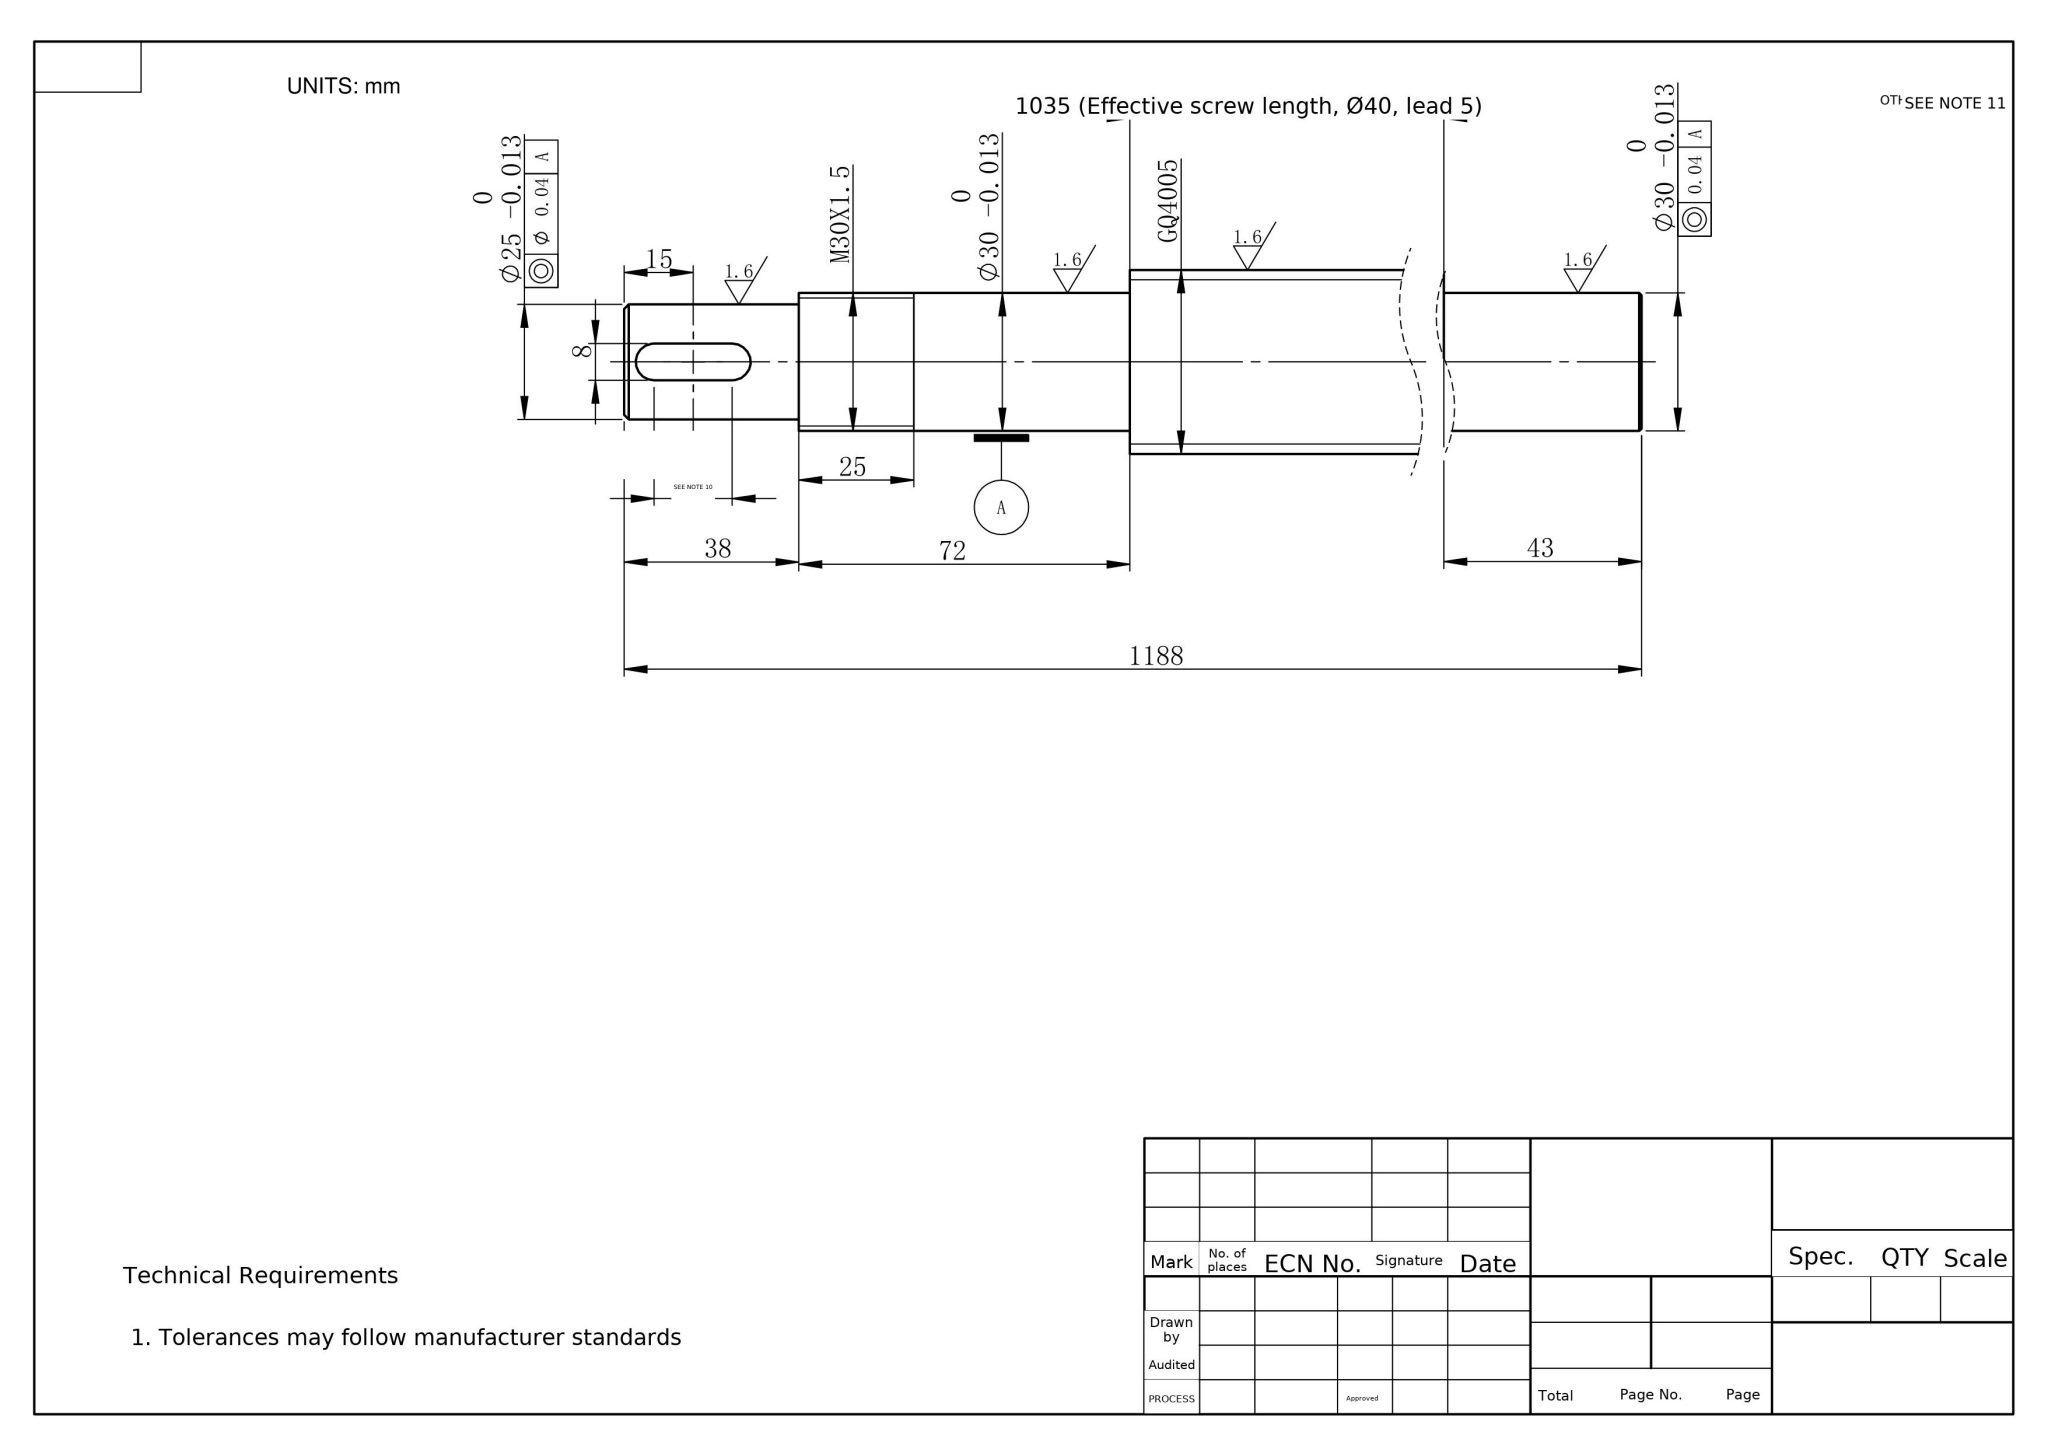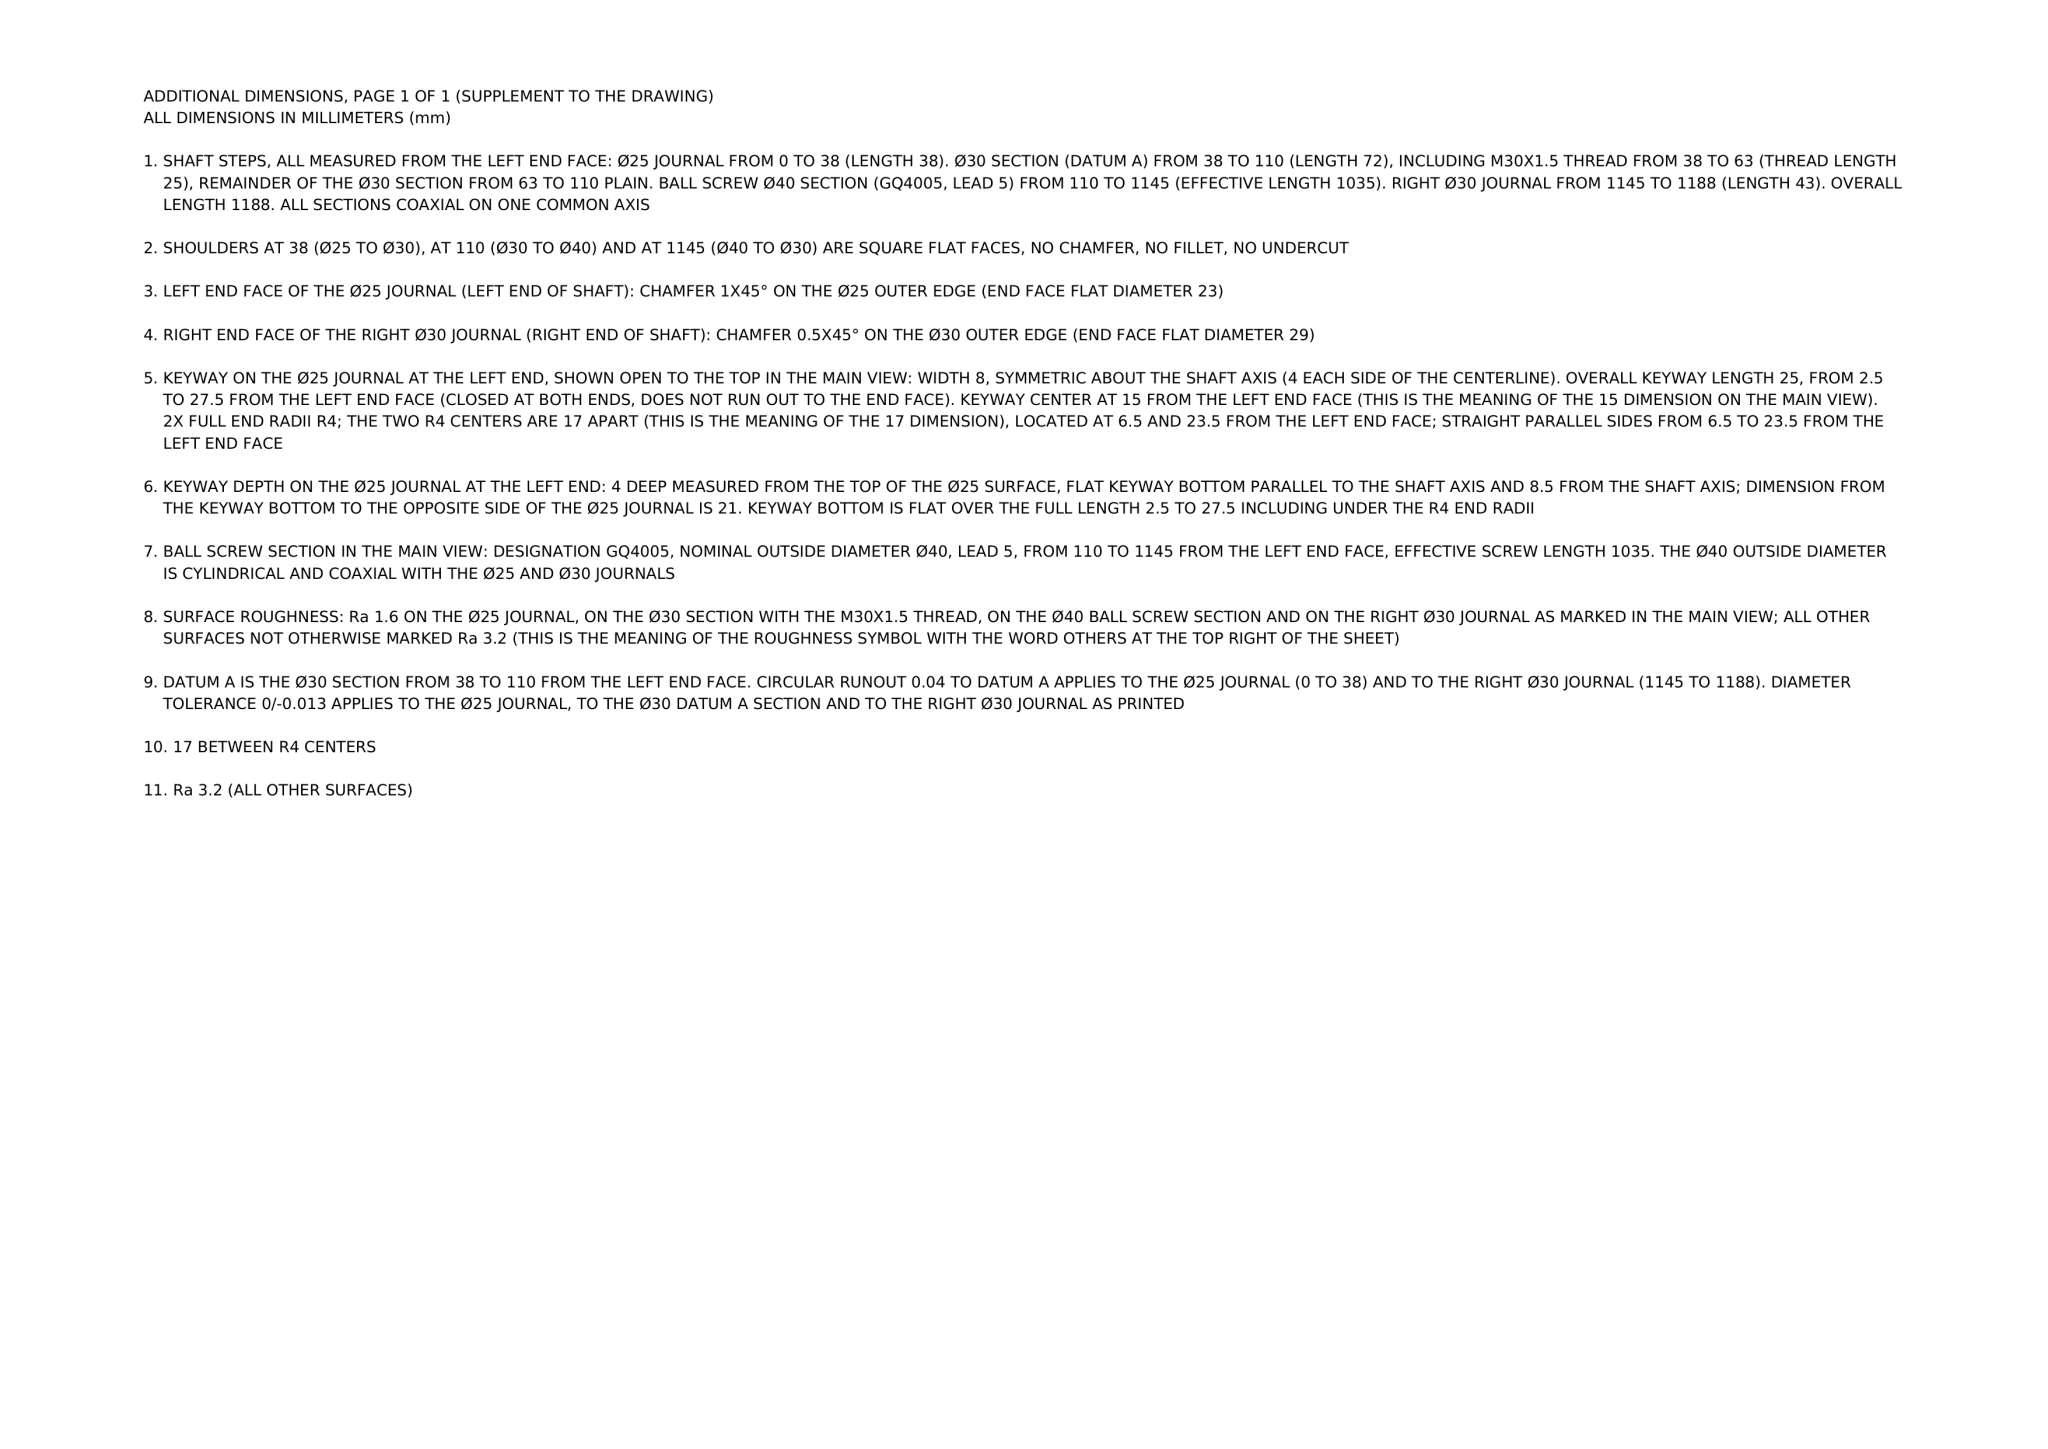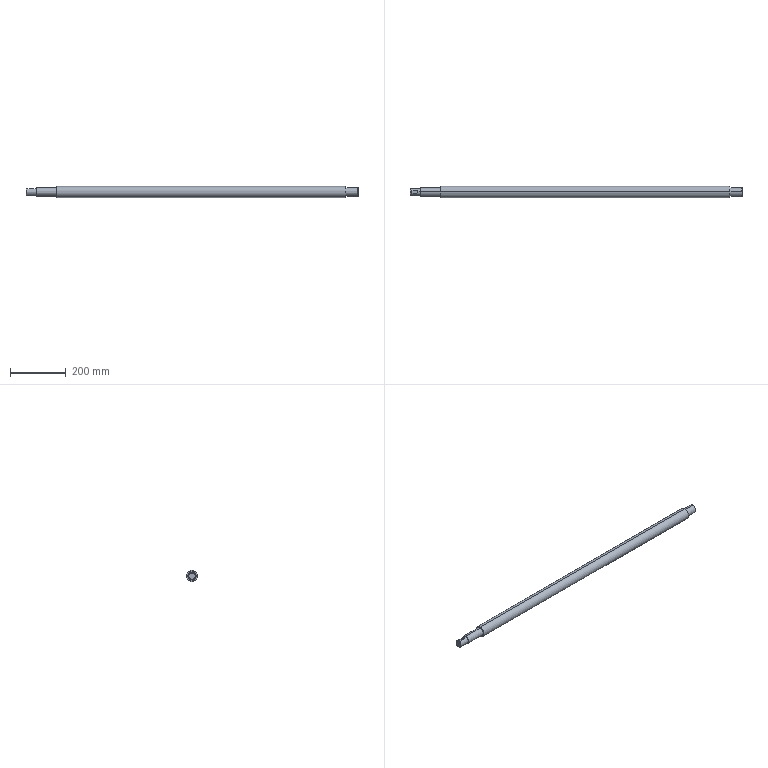Part | NX | mm | 1 solid | 23 faces | box 1188 x 40 x 40 mm | volume 1399804 mm3 | cylinder 11 | plane 8 | cone 4 | commonest cylinder face diameters 30 x4 8 x3 40 x2 25 x2
STEP:
#1=COLOUR_RGB('',1.,0.949,0.9098);
#2=FILL_AREA_STYLE_COLOUR('',#1);
#3=FILL_AREA_STYLE('',(#2));
#4=SURFACE_STYLE_FILL_AREA(#3);
#5=SURFACE_SIDE_STYLE('',(#4));
#6=SURFACE_STYLE_USAGE(.BOTH.,#5);
#7=PRESENTATION_STYLE_ASSIGNMENT((#6));
#8=CARTESIAN_POINT('',(110.,0.,-15.));
#9=VERTEX_POINT('',#8);
#10=CARTESIAN_POINT('',(38.,0.,-15.));
#11=VERTEX_POINT('',#10);
#12=CARTESIAN_POINT('',(0.,0.,-15.));
#13=DIRECTION('',(-1.,0.,0.));
#14=VECTOR('',#13,1000.);
#15=LINE('',#12,#14);
#16=EDGE_CURVE('',#9,#11,#15,.T.);
#17=ORIENTED_EDGE('',*,*,#16,.F.);
#18=CARTESIAN_POINT('',(110.,0.,15.));
#19=VERTEX_POINT('',#18);
#20=CARTESIAN_POINT('',(110.,0.,0.));
#21=DIRECTION('',(-1.,0.,0.));
#22=DIRECTION('',(0.,0.,1.));
#23=AXIS2_PLACEMENT_3D('',#20,#21,#22);
#24=CIRCLE('',#23,15.);
#25=EDGE_CURVE('',#9,#19,#24,.T.);
#26=ORIENTED_EDGE('',*,*,#25,.T.);
#27=CARTESIAN_POINT('',(38.,0.,15.));
#28=VERTEX_POINT('',#27);
#29=CARTESIAN_POINT('',(0.,0.,15.));
#30=DIRECTION('',(-1.,0.,0.));
#31=VECTOR('',#30,1000.);
#32=LINE('',#29,#31);
#33=EDGE_CURVE('',#19,#28,#32,.T.);
#34=ORIENTED_EDGE('',*,*,#33,.T.);
#35=CARTESIAN_POINT('',(38.,0.,0.));
#36=DIRECTION('',(-1.,0.,0.));
#37=DIRECTION('',(0.,0.,1.));
#38=AXIS2_PLACEMENT_3D('',#35,#36,#37);
#39=CIRCLE('',#38,15.);
#40=EDGE_CURVE('',#11,#28,#39,.T.);
#41=ORIENTED_EDGE('',*,*,#40,.F.);
#42=EDGE_LOOP('',(#17,#26,#34,#41));
#43=FACE_OUTER_BOUND('',#42,.T.);
#44=CARTESIAN_POINT('',(0.,0.,0.));
#45=DIRECTION('',(-1.,0.,0.));
#46=DIRECTION('',(0.,0.,1.));
#47=AXIS2_PLACEMENT_3D('',#44,#45,#46);
#48=CYLINDRICAL_SURFACE('',#47,15.);
#49=ADVANCED_FACE('',(#43),#48,.T.);
#50=STYLED_ITEM('',(#7),#49);
#51=(LENGTH_UNIT()NAMED_UNIT(*)SI_UNIT(.MILLI.,.METRE.));
#52=UNCERTAINTY_MEASURE_WITH_UNIT(LENGTH_MEASURE(0.00001),#51,'','');
#53=(NAMED_UNIT(*)PLANE_ANGLE_UNIT()SI_UNIT($,.RADIAN.));
#54=(NAMED_UNIT(*)SI_UNIT($,.STERADIAN.)SOLID_ANGLE_UNIT());
#55=(GEOMETRIC_REPRESENTATION_CONTEXT(3)GLOBAL_UNCERTAINTY_ASSIGNED_CONTEXT((#52))GLOBAL_UNIT_ASSIGNED_CONTEXT((#51,#53,#54))REPRESENTATION_CONTEXT('',''));
#56=MECHANICAL_DESIGN_GEOMETRIC_PRESENTATION_REPRESENTATION('',(#50),#55);
#57=PRESENTATION_LAYER_ASSIGNMENT('','',(#50));
#58=COLOUR_RGB('',1.,0.949,0.9098);
#59=FILL_AREA_STYLE_COLOUR('',#58);
#60=FILL_AREA_STYLE('',(#59));
#61=SURFACE_STYLE_FILL_AREA(#60);
#62=SURFACE_SIDE_STYLE('',(#61));
#63=SURFACE_STYLE_USAGE(.BOTH.,#62);
#64=PRESENTATION_STYLE_ASSIGNMENT((#63));
#65=CARTESIAN_POINT('',(1145.,0.,20.));
#66=VERTEX_POINT('',#65);
#67=CARTESIAN_POINT('',(1145.,0.,-20.));
#68=VERTEX_POINT('',#67);
#69=CARTESIAN_POINT('',(1145.,0.,0.));
#70=DIRECTION('',(-1.,0.,0.));
#71=DIRECTION('',(0.,0.,1.));
#72=AXIS2_PLACEMENT_3D('',#69,#70,#71);
#73=CIRCLE('',#72,20.);
#74=EDGE_CURVE('',#66,#68,#73,.T.);
#75=ORIENTED_EDGE('',*,*,#74,.T.);
#76=CARTESIAN_POINT('',(110.,0.,-20.));
#77=VERTEX_POINT('',#76);
#78=CARTESIAN_POINT('',(0.,0.,-20.));
#79=DIRECTION('',(-1.,0.,0.));
#80=VECTOR('',#79,1000.);
#81=LINE('',#78,#80);
#82=EDGE_CURVE('',#68,#77,#81,.T.);
#83=ORIENTED_EDGE('',*,*,#82,.T.);
#84=CARTESIAN_POINT('',(110.,0.,20.));
#85=VERTEX_POINT('',#84);
#86=CARTESIAN_POINT('',(110.,0.,0.));
#87=DIRECTION('',(-1.,0.,0.));
#88=DIRECTION('',(0.,0.,1.));
#89=AXIS2_PLACEMENT_3D('',#86,#87,#88);
#90=CIRCLE('',#89,20.);
#91=EDGE_CURVE('',#85,#77,#90,.T.);
#92=ORIENTED_EDGE('',*,*,#91,.F.);
#93=CARTESIAN_POINT('',(0.,0.,20.));
#94=DIRECTION('',(-1.,0.,0.));
#95=VECTOR('',#94,1000.);
#96=LINE('',#93,#95);
#97=EDGE_CURVE('',#66,#85,#96,.T.);
#98=ORIENTED_EDGE('',*,*,#97,.F.);
#99=EDGE_LOOP('',(#75,#83,#92,#98));
#100=FACE_OUTER_BOUND('',#99,.T.);
#101=CARTESIAN_POINT('',(0.,0.,0.));
#102=DIRECTION('',(-1.,0.,0.));
#103=DIRECTION('',(0.,0.,1.));
#104=AXIS2_PLACEMENT_3D('',#101,#102,#103);
#105=CYLINDRICAL_SURFACE('',#104,20.);
#106=ADVANCED_FACE('',(#100),#105,.T.);
#107=STYLED_ITEM('',(#64),#106);
#108=(LENGTH_UNIT()NAMED_UNIT(*)SI_UNIT(.MILLI.,.METRE.));
#109=UNCERTAINTY_MEASURE_WITH_UNIT(LENGTH_MEASURE(0.00001),#108,'','');
#110=(NAMED_UNIT(*)PLANE_ANGLE_UNIT()SI_UNIT($,.RADIAN.));
#111=(NAMED_UNIT(*)SI_UNIT($,.STERADIAN.)SOLID_ANGLE_UNIT());
#112=(GEOMETRIC_REPRESENTATION_CONTEXT(3)GLOBAL_UNCERTAINTY_ASSIGNED_CONTEXT((#109))GLOBAL_UNIT_ASSIGNED_CONTEXT((#108,#110,#111))REPRESENTATION_CONTEXT('',''));
#113=MECHANICAL_DESIGN_GEOMETRIC_PRESENTATION_REPRESENTATION('',(#107),#112);
#114=COLOUR_RGB('',1.,0.949,0.9098);
#115=FILL_AREA_STYLE_COLOUR('',#114);
#116=FILL_AREA_STYLE('',(#115));
#117=SURFACE_STYLE_FILL_AREA(#116);
#118=SURFACE_SIDE_STYLE('',(#117));
#119=SURFACE_STYLE_USAGE(.BOTH.,#118);
#120=PRESENTATION_STYLE_ASSIGNMENT((#119));
#121=ORIENTED_EDGE('',*,*,#82,.F.);
#122=CARTESIAN_POINT('',(1145.,0.,0.));
#123=DIRECTION('',(-1.,0.,0.));
#124=DIRECTION('',(0.,0.,1.));
#125=AXIS2_PLACEMENT_3D('',#122,#123,#124);
#126=CIRCLE('',#125,20.);
#127=EDGE_CURVE('',#68,#66,#126,.T.);
#128=ORIENTED_EDGE('',*,*,#127,.T.);
#129=ORIENTED_EDGE('',*,*,#97,.T.);
#130=CARTESIAN_POINT('',(110.,0.,0.));
#131=DIRECTION('',(-1.,0.,0.));
#132=DIRECTION('',(0.,0.,1.));
#133=AXIS2_PLACEMENT_3D('',#130,#131,#132);
#134=CIRCLE('',#133,20.);
#135=EDGE_CURVE('',#77,#85,#134,.T.);
#136=ORIENTED_EDGE('',*,*,#135,.F.);
#137=EDGE_LOOP('',(#121,#128,#129,#136));
#138=FACE_OUTER_BOUND('',#137,.T.);
#139=CARTESIAN_POINT('',(0.,0.,0.));
#140=DIRECTION('',(-1.,0.,0.));
#141=DIRECTION('',(0.,0.,1.));
#142=AXIS2_PLACEMENT_3D('',#139,#140,#141);
#143=CYLINDRICAL_SURFACE('',#142,20.);
#144=ADVANCED_FACE('',(#138),#143,.T.);
#145=STYLED_ITEM('',(#120),#144);
#146=(LENGTH_UNIT()NAMED_UNIT(*)SI_UNIT(.MILLI.,.METRE.));
#147=UNCERTAINTY_MEASURE_WITH_UNIT(LENGTH_MEASURE(0.00001),#146,'','');
#148=(NAMED_UNIT(*)PLANE_ANGLE_UNIT()SI_UNIT($,.RADIAN.));
#149=(NAMED_UNIT(*)SI_UNIT($,.STERADIAN.)SOLID_ANGLE_UNIT());
#150=(GEOMETRIC_REPRESENTATION_CONTEXT(3)GLOBAL_UNCERTAINTY_ASSIGNED_CONTEXT((#147))GLOBAL_UNIT_ASSIGNED_CONTEXT((#146,#148,#149))REPRESENTATION_CONTEXT('',''));
#151=MECHANICAL_DESIGN_GEOMETRIC_PRESENTATION_REPRESENTATION('',(#145),#150);
#152=PRESENTATION_LAYER_ASSIGNMENT('','',(#107));
#153=COLOUR_RGB('',1.,0.949,0.9098);
#154=FILL_AREA_STYLE_COLOUR('',#153);
#155=FILL_AREA_STYLE('',(#154));
#156=SURFACE_STYLE_FILL_AREA(#155);
#157=SURFACE_SIDE_STYLE('',(#156));
#158=SURFACE_STYLE_USAGE(.BOTH.,#157);
#159=PRESENTATION_STYLE_ASSIGNMENT((#158));
#160=CARTESIAN_POINT('',(27.5,0.,8.5));
#161=VERTEX_POINT('',#160);
#162=CARTESIAN_POINT('',(23.5,4.,8.5));
#163=VERTEX_POINT('',#162);
#164=CARTESIAN_POINT('',(23.5,0.,8.5));
#165=DIRECTION('',(0.,0.,1.));
#166=DIRECTION('',(1.,0.,0.));
#167=AXIS2_PLACEMENT_3D('',#164,#165,#166);
#168=CIRCLE('',#167,4.);
#169=EDGE_CURVE('',#161,#163,#168,.T.);
#170=ORIENTED_EDGE('',*,*,#169,.F.);
#171=CARTESIAN_POINT('',(27.5,0.,12.5));
#172=VERTEX_POINT('',#171);
#173=CARTESIAN_POINT('',(27.5,0.,8.5));
#174=DIRECTION('',(0.,0.,1.));
#175=VECTOR('',#174,1000.);
#176=LINE('',#173,#175);
#177=EDGE_CURVE('',#161,#172,#176,.T.);
#178=ORIENTED_EDGE('',*,*,#177,.T.);
#179=CARTESIAN_POINT('',(23.5,4.,11.843));
#180=VERTEX_POINT('',#179);
#181=CARTESIAN_POINT('',(23.5,4.,11.843));
#182=CARTESIAN_POINT('',(23.766,4.,11.843));
#183=CARTESIAN_POINT('',(24.028,3.974,11.852));
#184=CARTESIAN_POINT('',(24.541,3.871,11.886));
#185=CARTESIAN_POINT('',(24.796,3.793,11.911));
#186=CARTESIAN_POINT('',(25.28,3.592,11.973));
#187=CARTESIAN_POINT('',(25.509,3.469,12.01));
#188=CARTESIAN_POINT('',(25.943,3.178,12.09));
#189=CARTESIAN_POINT('',(26.146,3.011,12.134));
#190=CARTESIAN_POINT('',(26.513,2.644,12.219));
#191=CARTESIAN_POINT('',(26.678,2.444,12.261));
#192=CARTESIAN_POINT('',(26.97,2.006,12.34));
#193=CARTESIAN_POINT('',(27.093,1.776,12.375));
#194=CARTESIAN_POINT('',(27.293,1.295,12.435));
#195=CARTESIAN_POINT('',(27.371,1.041,12.459));
#196=CARTESIAN_POINT('',(27.474,0.5239,12.492));
#197=CARTESIAN_POINT('',(27.5,0.263,12.5));
#198=CARTESIAN_POINT('',(27.5,0.,12.5));
#199=B_SPLINE_CURVE_WITH_KNOTS('',3,(#181,#182,#183,#184,#185,#186,#187,#188,#189,#190,#191,#192,#193,#194,#195,#196,#197,#198),.UNSPECIFIED.,.F.,.F.,(4,2,2,2,2,2,2,2,4),(0.,0.000787,0.001574,0.002361,0.003148,0.003935,0.004722,0.005509,0.006296),.UNSPECIFIED.);
#200=EDGE_CURVE('',#180,#172,#199,.T.);
#201=ORIENTED_EDGE('',*,*,#200,.F.);
#202=CARTESIAN_POINT('',(23.5,4.,8.5));
#203=DIRECTION('',(0.,0.,1.));
#204=VECTOR('',#203,1000.);
#205=LINE('',#202,#204);
#206=EDGE_CURVE('',#163,#180,#205,.T.);
#207=ORIENTED_EDGE('',*,*,#206,.F.);
#208=EDGE_LOOP('',(#170,#178,#201,#207));
#209=FACE_OUTER_BOUND('',#208,.T.);
#210=CARTESIAN_POINT('',(23.5,0.,8.5));
#211=DIRECTION('',(0.,0.,1.));
#212=DIRECTION('',(1.,0.,0.));
#213=AXIS2_PLACEMENT_3D('',#210,#211,#212);
#214=CYLINDRICAL_SURFACE('',#213,4.);
#215=ADVANCED_FACE('',(#209),#214,.F.);
#216=CARTESIAN_POINT('',(1188.,0.,14.5));
#217=VERTEX_POINT('',#216);
#218=CARTESIAN_POINT('',(1188.,0.,-14.5));
#219=VERTEX_POINT('',#218);
#220=CARTESIAN_POINT('',(1188.,0.,0.));
#221=DIRECTION('',(-1.,0.,0.));
#222=DIRECTION('',(0.,0.,1.));
#223=AXIS2_PLACEMENT_3D('',#220,#221,#222);
#224=CIRCLE('',#223,14.5);
#225=EDGE_CURVE('',#217,#219,#224,.T.);
#226=ORIENTED_EDGE('',*,*,#225,.T.);
#227=CARTESIAN_POINT('',(1187.5,0.,-15.));
#228=VERTEX_POINT('',#227);
#229=CARTESIAN_POINT('',(1188.,0.,-14.5));
#230=DIRECTION('',(-0.7071,0.,-0.7071));
#231=VECTOR('',#230,1000.);
#232=LINE('',#229,#231);
#233=EDGE_CURVE('',#219,#228,#232,.T.);
#234=ORIENTED_EDGE('',*,*,#233,.T.);
#235=CARTESIAN_POINT('',(1187.5,0.,15.));
#236=VERTEX_POINT('',#235);
#237=CARTESIAN_POINT('',(1187.5,0.,0.));
#238=DIRECTION('',(-1.,0.,0.));
#239=DIRECTION('',(0.,0.,1.));
#240=AXIS2_PLACEMENT_3D('',#237,#238,#239);
#241=CIRCLE('',#240,15.);
#242=EDGE_CURVE('',#236,#228,#241,.T.);
#243=ORIENTED_EDGE('',*,*,#242,.F.);
#244=CARTESIAN_POINT('',(1188.,0.,14.5));
#245=DIRECTION('',(-0.7071,0.,0.7071));
#246=VECTOR('',#245,1000.);
#247=LINE('',#244,#246);
#248=EDGE_CURVE('',#217,#236,#247,.T.);
#249=ORIENTED_EDGE('',*,*,#248,.F.);
#250=EDGE_LOOP('',(#226,#234,#243,#249));
#251=FACE_OUTER_BOUND('',#250,.T.);
#252=CARTESIAN_POINT('',(1188.,0.,0.));
#253=DIRECTION('',(-1.,0.,0.));
#254=DIRECTION('',(0.,0.,1.));
#255=AXIS2_PLACEMENT_3D('',#252,#253,#254);
#256=CONICAL_SURFACE('',#255,14.5,0.7854);
#257=ADVANCED_FACE('',(#251),#256,.T.);
#258=ORIENTED_EDGE('',*,*,#242,.T.);
#259=CARTESIAN_POINT('',(1145.,0.,-15.));
#260=VERTEX_POINT('',#259);
#261=CARTESIAN_POINT('',(0.,0.,-15.));
#262=DIRECTION('',(-1.,0.,0.));
#263=VECTOR('',#262,1000.);
#264=LINE('',#261,#263);
#265=EDGE_CURVE('',#228,#260,#264,.T.);
#266=ORIENTED_EDGE('',*,*,#265,.T.);
#267=CARTESIAN_POINT('',(1145.,0.,15.));
#268=VERTEX_POINT('',#267);
#269=CARTESIAN_POINT('',(1145.,0.,0.));
#270=DIRECTION('',(-1.,0.,0.));
#271=DIRECTION('',(0.,0.,1.));
#272=AXIS2_PLACEMENT_3D('',#269,#270,#271);
#273=CIRCLE('',#272,15.);
#274=EDGE_CURVE('',#268,#260,#273,.T.);
#275=ORIENTED_EDGE('',*,*,#274,.F.);
#276=CARTESIAN_POINT('',(0.,0.,15.));
#277=DIRECTION('',(-1.,0.,0.));
#278=VECTOR('',#277,1000.);
#279=LINE('',#276,#278);
#280=EDGE_CURVE('',#236,#268,#279,.T.);
#281=ORIENTED_EDGE('',*,*,#280,.F.);
#282=EDGE_LOOP('',(#258,#266,#275,#281));
#283=FACE_OUTER_BOUND('',#282,.T.);
#284=CARTESIAN_POINT('',(0.,0.,0.));
#285=DIRECTION('',(-1.,0.,0.));
#286=DIRECTION('',(0.,0.,1.));
#287=AXIS2_PLACEMENT_3D('',#284,#285,#286);
#288=CYLINDRICAL_SURFACE('',#287,15.);
#289=ADVANCED_FACE('',(#283),#288,.T.);
#290=CARTESIAN_POINT('',(110.,0.,0.));
#291=DIRECTION('',(-1.,0.,0.));
#292=DIRECTION('',(0.,0.,1.));
#293=AXIS2_PLACEMENT_3D('',#290,#291,#292);
#294=CIRCLE('',#293,15.);
#295=EDGE_CURVE('',#19,#9,#294,.T.);
#296=ORIENTED_EDGE('',*,*,#295,.T.);
#297=ORIENTED_EDGE('',*,*,#16,.T.);
#298=CARTESIAN_POINT('',(38.,0.,0.));
#299=DIRECTION('',(-1.,0.,0.));
#300=DIRECTION('',(0.,0.,1.));
#301=AXIS2_PLACEMENT_3D('',#298,#299,#300);
#302=CIRCLE('',#301,15.);
#303=EDGE_CURVE('',#28,#11,#302,.T.);
#304=ORIENTED_EDGE('',*,*,#303,.F.);
#305=ORIENTED_EDGE('',*,*,#33,.F.);
#306=EDGE_LOOP('',(#296,#297,#304,#305));
#307=FACE_OUTER_BOUND('',#306,.T.);
#308=CARTESIAN_POINT('',(0.,0.,0.));
#309=DIRECTION('',(-1.,0.,0.));
#310=DIRECTION('',(0.,0.,1.));
#311=AXIS2_PLACEMENT_3D('',#308,#309,#310);
#312=CYLINDRICAL_SURFACE('',#311,15.);
#313=ADVANCED_FACE('',(#307),#312,.T.);
#314=CARTESIAN_POINT('',(38.,0.,12.5));
#315=VERTEX_POINT('',#314);
#316=CARTESIAN_POINT('',(38.,0.,-12.5));
#317=VERTEX_POINT('',#316);
#318=CARTESIAN_POINT('',(38.,0.,0.));
#319=DIRECTION('',(-1.,0.,0.));
#320=DIRECTION('',(0.,0.,1.));
#321=AXIS2_PLACEMENT_3D('',#318,#319,#320);
#322=CIRCLE('',#321,12.5);
#323=EDGE_CURVE('',#315,#317,#322,.T.);
#324=ORIENTED_EDGE('',*,*,#323,.T.);
#325=CARTESIAN_POINT('',(1.,0.,-12.5));
#326=VERTEX_POINT('',#325);
#327=CARTESIAN_POINT('',(0.,0.,-12.5));
#328=DIRECTION('',(-1.,0.,0.));
#329=VECTOR('',#328,1000.);
#330=LINE('',#327,#329);
#331=EDGE_CURVE('',#317,#326,#330,.T.);
#332=ORIENTED_EDGE('',*,*,#331,.T.);
#333=CARTESIAN_POINT('',(1.,0.,12.5));
#334=VERTEX_POINT('',#333);
#335=CARTESIAN_POINT('',(1.,0.,0.));
#336=DIRECTION('',(-1.,0.,0.));
#337=DIRECTION('',(0.,0.,1.));
#338=AXIS2_PLACEMENT_3D('',#335,#336,#337);
#339=CIRCLE('',#338,12.5);
#340=EDGE_CURVE('',#334,#326,#339,.T.);
#341=ORIENTED_EDGE('',*,*,#340,.F.);
#342=CARTESIAN_POINT('',(2.5,-0.,12.5));
#343=VERTEX_POINT('',#342);
#344=CARTESIAN_POINT('',(0.,0.,12.5));
#345=DIRECTION('',(-1.,0.,0.));
#346=VECTOR('',#345,1000.);
#347=LINE('',#344,#346);
#348=EDGE_CURVE('',#343,#334,#347,.T.);
#349=ORIENTED_EDGE('',*,*,#348,.F.);
#350=CARTESIAN_POINT('',(6.5,4.,11.843));
#351=VERTEX_POINT('',#350);
#352=CARTESIAN_POINT('',(2.5,-0.,12.5));
#353=CARTESIAN_POINT('',(2.5,0.2627,12.5));
#354=CARTESIAN_POINT('',(2.527,0.5294,12.491));
#355=CARTESIAN_POINT('',(2.63,1.043,12.459));
#356=CARTESIAN_POINT('',(2.706,1.293,12.435));
#357=CARTESIAN_POINT('',(2.908,1.78,12.375));
#358=CARTESIAN_POINT('',(3.032,2.011,12.339));
#359=CARTESIAN_POINT('',(3.321,2.442,12.261));
#360=CARTESIAN_POINT('',(3.488,2.645,12.218));
#361=CARTESIAN_POINT('',(3.856,3.013,12.133));
#362=CARTESIAN_POINT('',(4.056,3.177,12.09));
#363=CARTESIAN_POINT('',(4.488,3.467,12.011));
#364=CARTESIAN_POINT('',(4.722,3.592,11.973));
#365=CARTESIAN_POINT('',(5.203,3.793,11.911));
#366=CARTESIAN_POINT('',(5.452,3.869,11.886));
#367=CARTESIAN_POINT('',(5.968,3.973,11.852));
#368=CARTESIAN_POINT('',(6.234,4.,11.843));
#369=CARTESIAN_POINT('',(6.5,4.,11.843));
#370=B_SPLINE_CURVE_WITH_KNOTS('',3,(#352,#353,#354,#355,#356,#357,#358,#359,#360,#361,#362,#363,#364,#365,#366,#367,#368,#369),.UNSPECIFIED.,.F.,.F.,(4,2,2,2,2,2,2,2,4),(0.006296,0.007082,0.007868,0.008654,0.00944,0.01023,0.01101,0.0118,0.01258),.UNSPECIFIED.);
#371=EDGE_CURVE('',#343,#351,#370,.T.);
#372=ORIENTED_EDGE('',*,*,#371,.T.);
#373=CARTESIAN_POINT('',(-0.,4.,11.843));
#374=DIRECTION('',(1.,0.,0.));
#375=VECTOR('',#374,1000.);
#376=LINE('',#373,#375);
#377=EDGE_CURVE('',#351,#180,#376,.T.);
#378=ORIENTED_EDGE('',*,*,#377,.T.);
#379=ORIENTED_EDGE('',*,*,#200,.T.);
#380=CARTESIAN_POINT('',(0.,0.,12.5));
#381=DIRECTION('',(-1.,0.,0.));
#382=VECTOR('',#381,1000.);
#383=LINE('',#380,#382);
#384=EDGE_CURVE('',#315,#172,#383,.T.);
#385=ORIENTED_EDGE('',*,*,#384,.F.);
#386=EDGE_LOOP('',(#324,#332,#341,#349,#372,#378,#379,#385));
#387=FACE_OUTER_BOUND('',#386,.T.);
#388=CARTESIAN_POINT('',(0.,0.,0.));
#389=DIRECTION('',(-1.,0.,0.));
#390=DIRECTION('',(0.,0.,1.));
#391=AXIS2_PLACEMENT_3D('',#388,#389,#390);
#392=CYLINDRICAL_SURFACE('',#391,12.5);
#393=ADVANCED_FACE('',(#387),#392,.T.);
#394=CARTESIAN_POINT('',(0.,0.,11.5));
#395=VERTEX_POINT('',#394);
#396=CARTESIAN_POINT('',(0.,0.,-11.5));
#397=VERTEX_POINT('',#396);
#398=CARTESIAN_POINT('',(0.,0.,0.));
#399=DIRECTION('',(-1.,0.,0.));
#400=DIRECTION('',(0.,0.,1.));
#401=AXIS2_PLACEMENT_3D('',#398,#399,#400);
#402=CIRCLE('',#401,11.5);
#403=EDGE_CURVE('',#395,#397,#402,.T.);
#404=ORIENTED_EDGE('',*,*,#403,.F.);
#405=CARTESIAN_POINT('',(1.,0.,12.5));
#406=DIRECTION('',(0.7071,0.,0.7071));
#407=VECTOR('',#406,1000.);
#408=LINE('',#405,#407);
#409=EDGE_CURVE('',#395,#334,#408,.T.);
#410=ORIENTED_EDGE('',*,*,#409,.T.);
#411=ORIENTED_EDGE('',*,*,#340,.T.);
#412=CARTESIAN_POINT('',(1.,0.,-12.5));
#413=DIRECTION('',(0.7071,0.,-0.7071));
#414=VECTOR('',#413,1000.);
#415=LINE('',#412,#414);
#416=EDGE_CURVE('',#397,#326,#415,.T.);
#417=ORIENTED_EDGE('',*,*,#416,.F.);
#418=EDGE_LOOP('',(#404,#410,#411,#417));
#419=FACE_OUTER_BOUND('',#418,.T.);
#420=CARTESIAN_POINT('',(1.,0.,0.));
#421=DIRECTION('',(1.,0.,0.));
#422=DIRECTION('',(0.,0.,-1.));
#423=AXIS2_PLACEMENT_3D('',#420,#421,#422);
#424=CONICAL_SURFACE('',#423,12.5,0.7854);
#425=ADVANCED_FACE('',(#419),#424,.T.);
#426=CARTESIAN_POINT('',(0.,0.,0.));
#427=DIRECTION('',(-1.,0.,0.));
#428=DIRECTION('',(0.,0.,1.));
#429=AXIS2_PLACEMENT_3D('',#426,#427,#428);
#430=CIRCLE('',#429,11.5);
#431=EDGE_CURVE('',#397,#395,#430,.T.);
#432=ORIENTED_EDGE('',*,*,#431,.T.);
#433=ORIENTED_EDGE('',*,*,#403,.T.);
#434=EDGE_LOOP('',(#432,#433));
#435=FACE_OUTER_BOUND('',#434,.T.);
#436=CARTESIAN_POINT('',(0.,0.,0.));
#437=DIRECTION('',(1.,0.,0.));
#438=DIRECTION('',(0.,0.,-1.));
#439=AXIS2_PLACEMENT_3D('',#436,#437,#438);
#440=PLANE('',#439);
#441=ADVANCED_FACE('',(#435),#440,.F.);
#442=ORIENTED_EDGE('',*,*,#409,.F.);
#443=ORIENTED_EDGE('',*,*,#431,.F.);
#444=ORIENTED_EDGE('',*,*,#416,.T.);
#445=CARTESIAN_POINT('',(1.,0.,0.));
#446=DIRECTION('',(-1.,0.,0.));
#447=DIRECTION('',(0.,0.,1.));
#448=AXIS2_PLACEMENT_3D('',#445,#446,#447);
#449=CIRCLE('',#448,12.5);
#450=EDGE_CURVE('',#326,#334,#449,.T.);
#451=ORIENTED_EDGE('',*,*,#450,.T.);
#452=EDGE_LOOP('',(#442,#443,#444,#451));
#453=FACE_OUTER_BOUND('',#452,.T.);
#454=CARTESIAN_POINT('',(1.,0.,0.));
#455=DIRECTION('',(1.,0.,0.));
#456=DIRECTION('',(0.,0.,-1.));
#457=AXIS2_PLACEMENT_3D('',#454,#455,#456);
#458=CONICAL_SURFACE('',#457,12.5,0.7854);
#459=ADVANCED_FACE('',(#453),#458,.T.);
#460=ORIENTED_EDGE('',*,*,#331,.F.);
#461=CARTESIAN_POINT('',(38.,0.,0.));
#462=DIRECTION('',(-1.,0.,0.));
#463=DIRECTION('',(0.,0.,1.));
#464=AXIS2_PLACEMENT_3D('',#461,#462,#463);
#465=CIRCLE('',#464,12.5);
#466=EDGE_CURVE('',#317,#315,#465,.T.);
#467=ORIENTED_EDGE('',*,*,#466,.T.);
#468=ORIENTED_EDGE('',*,*,#384,.T.);
#469=CARTESIAN_POINT('',(23.5,-4.,11.843));
#470=VERTEX_POINT('',#469);
#471=CARTESIAN_POINT('',(27.5,0.,12.5));
#472=CARTESIAN_POINT('',(27.5,-0.2627,12.5));
#473=CARTESIAN_POINT('',(27.473,-0.5294,12.491));
#474=CARTESIAN_POINT('',(27.37,-1.043,12.459));
#475=CARTESIAN_POINT('',(27.294,-1.293,12.435));
#476=CARTESIAN_POINT('',(27.092,-1.78,12.375));
#477=CARTESIAN_POINT('',(26.968,-2.011,12.339));
#478=CARTESIAN_POINT('',(26.679,-2.442,12.261));
#479=CARTESIAN_POINT('',(26.512,-2.645,12.218));
#480=CARTESIAN_POINT('',(26.144,-3.013,12.133));
#481=CARTESIAN_POINT('',(25.944,-3.177,12.09));
#482=CARTESIAN_POINT('',(25.512,-3.467,12.011));
#483=CARTESIAN_POINT('',(25.278,-3.592,11.973));
#484=CARTESIAN_POINT('',(24.797,-3.793,11.911));
#485=CARTESIAN_POINT('',(24.548,-3.869,11.886));
#486=CARTESIAN_POINT('',(24.032,-3.973,11.852));
#487=CARTESIAN_POINT('',(23.766,-4.,11.843));
#488=CARTESIAN_POINT('',(23.5,-4.,11.843));
#489=B_SPLINE_CURVE_WITH_KNOTS('',3,(#471,#472,#473,#474,#475,#476,#477,#478,#479,#480,#481,#482,#483,#484,#485,#486,#487,#488),.UNSPECIFIED.,.F.,.F.,(4,2,2,2,2,2,2,2,4),(0.006296,0.007082,0.007868,0.008654,0.00944,0.01023,0.01101,0.0118,0.01258),.UNSPECIFIED.);
#490=EDGE_CURVE('',#172,#470,#489,.T.);
#491=ORIENTED_EDGE('',*,*,#490,.T.);
#492=CARTESIAN_POINT('',(6.5,-4.,11.843));
#493=VERTEX_POINT('',#492);
#494=CARTESIAN_POINT('',(0.,-4.,11.843));
#495=DIRECTION('',(-1.,0.,0.));
#496=VECTOR('',#495,1000.);
#497=LINE('',#494,#496);
#498=EDGE_CURVE('',#470,#493,#497,.T.);
#499=ORIENTED_EDGE('',*,*,#498,.T.);
#500=CARTESIAN_POINT('',(6.5,-4.,11.843));
#501=CARTESIAN_POINT('',(6.234,-4.,11.843));
#502=CARTESIAN_POINT('',(5.972,-3.974,11.852));
#503=CARTESIAN_POINT('',(5.459,-3.871,11.886));
#504=CARTESIAN_POINT('',(5.204,-3.793,11.911));
#505=CARTESIAN_POINT('',(4.72,-3.592,11.973));
#506=CARTESIAN_POINT('',(4.491,-3.469,12.01));
#507=CARTESIAN_POINT('',(4.057,-3.178,12.09));
#508=CARTESIAN_POINT('',(3.854,-3.011,12.134));
#509=CARTESIAN_POINT('',(3.487,-2.644,12.219));
#510=CARTESIAN_POINT('',(3.322,-2.444,12.261));
#511=CARTESIAN_POINT('',(3.03,-2.006,12.34));
#512=CARTESIAN_POINT('',(2.907,-1.776,12.375));
#513=CARTESIAN_POINT('',(2.707,-1.295,12.435));
#514=CARTESIAN_POINT('',(2.629,-1.041,12.459));
#515=CARTESIAN_POINT('',(2.526,-0.5239,12.492));
#516=CARTESIAN_POINT('',(2.5,-0.263,12.5));
#517=CARTESIAN_POINT('',(2.5,-0.,12.5));
#518=B_SPLINE_CURVE_WITH_KNOTS('',3,(#500,#501,#502,#503,#504,#505,#506,#507,#508,#509,#510,#511,#512,#513,#514,#515,#516,#517),.UNSPECIFIED.,.F.,.F.,(4,2,2,2,2,2,2,2,4),(0.,0.000787,0.001574,0.002361,0.003148,0.003935,0.004722,0.005509,0.006296),.UNSPECIFIED.);
#519=EDGE_CURVE('',#493,#343,#518,.T.);
#520=ORIENTED_EDGE('',*,*,#519,.T.);
#521=ORIENTED_EDGE('',*,*,#348,.T.);
#522=ORIENTED_EDGE('',*,*,#450,.F.);
#523=EDGE_LOOP('',(#460,#467,#468,#491,#499,#520,#521,#522));
#524=FACE_OUTER_BOUND('',#523,.T.);
#525=CARTESIAN_POINT('',(0.,0.,0.));
#526=DIRECTION('',(-1.,0.,0.));
#527=DIRECTION('',(0.,0.,1.));
#528=AXIS2_PLACEMENT_3D('',#525,#526,#527);
#529=CYLINDRICAL_SURFACE('',#528,12.5);
#530=ADVANCED_FACE('',(#524),#529,.T.);
#531=ORIENTED_EDGE('',*,*,#323,.F.);
#532=ORIENTED_EDGE('',*,*,#466,.F.);
#533=EDGE_LOOP('',(#531,#532));
#534=FACE_BOUND('',#533,.T.);
#535=ORIENTED_EDGE('',*,*,#303,.T.);
#536=ORIENTED_EDGE('',*,*,#40,.T.);
#537=EDGE_LOOP('',(#535,#536));
#538=FACE_OUTER_BOUND('',#537,.T.);
#539=CARTESIAN_POINT('',(38.,12.5,0.));
#540=DIRECTION('',(1.,0.,0.));
#541=DIRECTION('',(0.,0.,-1.));
#542=AXIS2_PLACEMENT_3D('',#539,#540,#541);
#543=PLANE('',#542);
#544=ADVANCED_FACE('',(#534,#538),#543,.F.);
#545=ORIENTED_EDGE('',*,*,#295,.F.);
#546=ORIENTED_EDGE('',*,*,#25,.F.);
#547=EDGE_LOOP('',(#545,#546));
#548=FACE_BOUND('',#547,.T.);
#549=ORIENTED_EDGE('',*,*,#91,.T.);
#550=ORIENTED_EDGE('',*,*,#135,.T.);
#551=EDGE_LOOP('',(#549,#550));
#552=FACE_OUTER_BOUND('',#551,.T.);
#553=CARTESIAN_POINT('',(110.,15.,0.));
#554=DIRECTION('',(1.,0.,0.));
#555=DIRECTION('',(0.,0.,-1.));
#556=AXIS2_PLACEMENT_3D('',#553,#554,#555);
#557=PLANE('',#556);
#558=ADVANCED_FACE('',(#548,#552),#557,.F.);
#559=ORIENTED_EDGE('',*,*,#74,.F.);
#560=ORIENTED_EDGE('',*,*,#127,.F.);
#561=EDGE_LOOP('',(#559,#560));
#562=FACE_OUTER_BOUND('',#561,.T.);
#563=ORIENTED_EDGE('',*,*,#274,.T.);
#564=CARTESIAN_POINT('',(1145.,0.,0.));
#565=DIRECTION('',(-1.,0.,0.));
#566=DIRECTION('',(0.,0.,1.));
#567=AXIS2_PLACEMENT_3D('',#564,#565,#566);
#568=CIRCLE('',#567,15.);
#569=EDGE_CURVE('',#260,#268,#568,.T.);
#570=ORIENTED_EDGE('',*,*,#569,.T.);
#571=EDGE_LOOP('',(#563,#570));
#572=FACE_BOUND('',#571,.T.);
#573=CARTESIAN_POINT('',(1145.,20.,0.));
#574=DIRECTION('',(-1.,0.,0.));
#575=DIRECTION('',(0.,0.,1.));
#576=AXIS2_PLACEMENT_3D('',#573,#574,#575);
#577=PLANE('',#576);
#578=ADVANCED_FACE('',(#562,#572),#577,.F.);
#579=ORIENTED_EDGE('',*,*,#265,.F.);
#580=CARTESIAN_POINT('',(1187.5,0.,0.));
#581=DIRECTION('',(-1.,0.,0.));
#582=DIRECTION('',(0.,0.,1.));
#583=AXIS2_PLACEMENT_3D('',#580,#581,#582);
#584=CIRCLE('',#583,15.);
#585=EDGE_CURVE('',#228,#236,#584,.T.);
#586=ORIENTED_EDGE('',*,*,#585,.T.);
#587=ORIENTED_EDGE('',*,*,#280,.T.);
#588=ORIENTED_EDGE('',*,*,#569,.F.);
#589=EDGE_LOOP('',(#579,#586,#587,#588));
#590=FACE_OUTER_BOUND('',#589,.T.);
#591=CARTESIAN_POINT('',(0.,0.,0.));
#592=DIRECTION('',(-1.,0.,0.));
#593=DIRECTION('',(0.,0.,1.));
#594=AXIS2_PLACEMENT_3D('',#591,#592,#593);
#595=CYLINDRICAL_SURFACE('',#594,15.);
#596=ADVANCED_FACE('',(#590),#595,.T.);
#597=ORIENTED_EDGE('',*,*,#233,.F.);
#598=CARTESIAN_POINT('',(1188.,0.,0.));
#599=DIRECTION('',(-1.,0.,0.));
#600=DIRECTION('',(0.,0.,1.));
#601=AXIS2_PLACEMENT_3D('',#598,#599,#600);
#602=CIRCLE('',#601,14.5);
#603=EDGE_CURVE('',#219,#217,#602,.T.);
#604=ORIENTED_EDGE('',*,*,#603,.T.);
#605=ORIENTED_EDGE('',*,*,#248,.T.);
#606=ORIENTED_EDGE('',*,*,#585,.F.);
#607=EDGE_LOOP('',(#597,#604,#605,#606));
#608=FACE_OUTER_BOUND('',#607,.T.);
#609=CARTESIAN_POINT('',(1188.,0.,0.));
#610=DIRECTION('',(-1.,0.,0.));
#611=DIRECTION('',(0.,0.,1.));
#612=AXIS2_PLACEMENT_3D('',#609,#610,#611);
#613=CONICAL_SURFACE('',#612,14.5,0.7854);
#614=ADVANCED_FACE('',(#608),#613,.T.);
#615=ORIENTED_EDGE('',*,*,#225,.F.);
#616=ORIENTED_EDGE('',*,*,#603,.F.);
#617=EDGE_LOOP('',(#615,#616));
#618=FACE_OUTER_BOUND('',#617,.T.);
#619=CARTESIAN_POINT('',(1188.,14.5,0.));
#620=DIRECTION('',(-1.,0.,0.));
#621=DIRECTION('',(0.,0.,1.));
#622=AXIS2_PLACEMENT_3D('',#619,#620,#621);
#623=PLANE('',#622);
#624=ADVANCED_FACE('',(#618),#623,.F.);
#625=CARTESIAN_POINT('',(6.5,-4.,8.5));
#626=VERTEX_POINT('',#625);
#627=CARTESIAN_POINT('',(6.5,-4.,8.5));
#628=DIRECTION('',(0.,0.,1.));
#629=VECTOR('',#628,1000.);
#630=LINE('',#627,#629);
#631=EDGE_CURVE('',#626,#493,#630,.T.);
#632=ORIENTED_EDGE('',*,*,#631,.F.);
#633=CARTESIAN_POINT('',(6.5,4.,8.5));
#634=VERTEX_POINT('',#633);
#635=CARTESIAN_POINT('',(6.5,0.,8.5));
#636=DIRECTION('',(0.,0.,1.));
#637=DIRECTION('',(1.,0.,0.));
#638=AXIS2_PLACEMENT_3D('',#635,#636,#637);
#639=CIRCLE('',#638,4.);
#640=EDGE_CURVE('',#634,#626,#639,.T.);
#641=ORIENTED_EDGE('',*,*,#640,.F.);
#642=CARTESIAN_POINT('',(6.5,4.,8.5));
#643=DIRECTION('',(0.,0.,1.));
#644=VECTOR('',#643,1000.);
#645=LINE('',#642,#644);
#646=EDGE_CURVE('',#634,#351,#645,.T.);
#647=ORIENTED_EDGE('',*,*,#646,.T.);
#648=ORIENTED_EDGE('',*,*,#371,.F.);
#649=ORIENTED_EDGE('',*,*,#519,.F.);
#650=EDGE_LOOP('',(#632,#641,#647,#648,#649));
#651=FACE_OUTER_BOUND('',#650,.T.);
#652=CARTESIAN_POINT('',(6.5,0.,8.5));
#653=DIRECTION('',(0.,0.,1.));
#654=DIRECTION('',(1.,0.,0.));
#655=AXIS2_PLACEMENT_3D('',#652,#653,#654);
#656=CYLINDRICAL_SURFACE('',#655,4.);
#657=ADVANCED_FACE('',(#651),#656,.F.);
#658=ORIENTED_EDGE('',*,*,#646,.F.);
#659=CARTESIAN_POINT('',(6.5,4.,8.5));
#660=DIRECTION('',(-1.,-0.,0.));
#661=VECTOR('',#660,1000.);
#662=LINE('',#659,#661);
#663=EDGE_CURVE('',#163,#634,#662,.T.);
#664=ORIENTED_EDGE('',*,*,#663,.F.);
#665=ORIENTED_EDGE('',*,*,#206,.T.);
#666=ORIENTED_EDGE('',*,*,#377,.F.);
#667=EDGE_LOOP('',(#658,#664,#665,#666));
#668=FACE_OUTER_BOUND('',#667,.T.);
#669=CARTESIAN_POINT('',(6.5,4.,8.5));
#670=DIRECTION('',(-0.,1.,0.));
#671=DIRECTION('',(-1.,-0.,0.));
#672=AXIS2_PLACEMENT_3D('',#669,#670,#671);
#673=PLANE('',#672);
#674=ADVANCED_FACE('',(#668),#673,.F.);
#675=ORIENTED_EDGE('',*,*,#177,.F.);
#676=CARTESIAN_POINT('',(23.5,-4.,8.5));
#677=VERTEX_POINT('',#676);
#678=CARTESIAN_POINT('',(23.5,0.,8.5));
#679=DIRECTION('',(0.,0.,1.));
#680=DIRECTION('',(1.,0.,0.));
#681=AXIS2_PLACEMENT_3D('',#678,#679,#680);
#682=CIRCLE('',#681,4.);
#683=EDGE_CURVE('',#677,#161,#682,.T.);
#684=ORIENTED_EDGE('',*,*,#683,.F.);
#685=CARTESIAN_POINT('',(23.5,-4.,8.5));
#686=DIRECTION('',(0.,0.,1.));
#687=VECTOR('',#686,1000.);
#688=LINE('',#685,#687);
#689=EDGE_CURVE('',#677,#470,#688,.T.);
#690=ORIENTED_EDGE('',*,*,#689,.T.);
#691=ORIENTED_EDGE('',*,*,#490,.F.);
#692=EDGE_LOOP('',(#675,#684,#690,#691));
#693=FACE_OUTER_BOUND('',#692,.T.);
#694=CARTESIAN_POINT('',(23.5,0.,8.5));
#695=DIRECTION('',(0.,0.,1.));
#696=DIRECTION('',(1.,0.,0.));
#697=AXIS2_PLACEMENT_3D('',#694,#695,#696);
#698=CYLINDRICAL_SURFACE('',#697,4.);
#699=ADVANCED_FACE('',(#693),#698,.F.);
#700=ORIENTED_EDGE('',*,*,#689,.F.);
#701=CARTESIAN_POINT('',(6.5,-4.,8.5));
#702=DIRECTION('',(1.,0.,0.));
#703=VECTOR('',#702,1000.);
#704=LINE('',#701,#703);
#705=EDGE_CURVE('',#626,#677,#704,.T.);
#706=ORIENTED_EDGE('',*,*,#705,.F.);
#707=ORIENTED_EDGE('',*,*,#631,.T.);
#708=ORIENTED_EDGE('',*,*,#498,.F.);
#709=EDGE_LOOP('',(#700,#706,#707,#708));
#710=FACE_OUTER_BOUND('',#709,.T.);
#711=CARTESIAN_POINT('',(6.5,-4.,8.5));
#712=DIRECTION('',(0.,-1.,0.));
#713=DIRECTION('',(1.,0.,0.));
#714=AXIS2_PLACEMENT_3D('',#711,#712,#713);
#715=PLANE('',#714);
#716=ADVANCED_FACE('',(#710),#715,.F.);
#717=ORIENTED_EDGE('',*,*,#640,.T.);
#718=ORIENTED_EDGE('',*,*,#705,.T.);
#719=ORIENTED_EDGE('',*,*,#683,.T.);
#720=ORIENTED_EDGE('',*,*,#169,.T.);
#721=ORIENTED_EDGE('',*,*,#663,.T.);
#722=EDGE_LOOP('',(#717,#718,#719,#720,#721));
#723=FACE_OUTER_BOUND('',#722,.T.);
#724=CARTESIAN_POINT('',(6.5,0.,8.5));
#725=DIRECTION('',(0.,0.,1.));
#726=DIRECTION('',(1.,0.,0.));
#727=AXIS2_PLACEMENT_3D('',#724,#725,#726);
#728=PLANE('',#727);
#729=ADVANCED_FACE('',(#723),#728,.T.);
#730=CLOSED_SHELL('',(#215,#257,#289,#106,#313,#393,#425,#441,#459,#530,#544,#49,#558,#144,#578,#596,#614,#624,#657,#674,#699,#716,#729));
#731=MANIFOLD_SOLID_BREP('',#730);
#732=CARTESIAN_POINT('',(0.,0.,0.));
#733=DIRECTION('',(0.,0.,1.));
#734=DIRECTION('',(1.,0.,0.));
#735=AXIS2_PLACEMENT_3D('',#732,#733,#734);
#736=(LENGTH_UNIT()NAMED_UNIT(*)SI_UNIT(.MILLI.,.METRE.));
#737=UNCERTAINTY_MEASURE_WITH_UNIT(LENGTH_MEASURE(0.00001),#736,'','');
#738=(NAMED_UNIT(*)PLANE_ANGLE_UNIT()SI_UNIT($,.RADIAN.));
#739=(NAMED_UNIT(*)SI_UNIT($,.STERADIAN.)SOLID_ANGLE_UNIT());
#740=(GEOMETRIC_REPRESENTATION_CONTEXT(3)GLOBAL_UNCERTAINTY_ASSIGNED_CONTEXT((#737))GLOBAL_UNIT_ASSIGNED_CONTEXT((#736,#738,#739))REPRESENTATION_CONTEXT('',''));
#741=ADVANCED_BREP_SHAPE_REPRESENTATION('',(#731,#735),#740);
#742=STYLED_ITEM('',(#159),#741);
#743=(LENGTH_UNIT()NAMED_UNIT(*)SI_UNIT(.MILLI.,.METRE.));
#744=UNCERTAINTY_MEASURE_WITH_UNIT(LENGTH_MEASURE(0.00001),#743,'','');
#745=(NAMED_UNIT(*)PLANE_ANGLE_UNIT()SI_UNIT($,.RADIAN.));
#746=(NAMED_UNIT(*)SI_UNIT($,.STERADIAN.)SOLID_ANGLE_UNIT());
#747=(GEOMETRIC_REPRESENTATION_CONTEXT(3)GLOBAL_UNCERTAINTY_ASSIGNED_CONTEXT((#744))GLOBAL_UNIT_ASSIGNED_CONTEXT((#743,#745,#746))REPRESENTATION_CONTEXT('',''));
#748=MECHANICAL_DESIGN_GEOMETRIC_PRESENTATION_REPRESENTATION('',(#742),#747);
#749=COLOUR_RGB('',1.,0.949,0.9098);
#750=FILL_AREA_STYLE_COLOUR('',#749);
#751=FILL_AREA_STYLE('',(#750));
#752=SURFACE_STYLE_FILL_AREA(#751);
#753=SURFACE_SIDE_STYLE('',(#752));
#754=SURFACE_STYLE_USAGE(.BOTH.,#753);
#755=PRESENTATION_STYLE_ASSIGNMENT((#754));
#756=STYLED_ITEM('',(#755),#313);
#757=(LENGTH_UNIT()NAMED_UNIT(*)SI_UNIT(.MILLI.,.METRE.));
#758=UNCERTAINTY_MEASURE_WITH_UNIT(LENGTH_MEASURE(0.00001),#757,'','');
#759=(NAMED_UNIT(*)PLANE_ANGLE_UNIT()SI_UNIT($,.RADIAN.));
#760=(NAMED_UNIT(*)SI_UNIT($,.STERADIAN.)SOLID_ANGLE_UNIT());
#761=(GEOMETRIC_REPRESENTATION_CONTEXT(3)GLOBAL_UNCERTAINTY_ASSIGNED_CONTEXT((#758))GLOBAL_UNIT_ASSIGNED_CONTEXT((#757,#759,#760))REPRESENTATION_CONTEXT('',''));
#762=MECHANICAL_DESIGN_GEOMETRIC_PRESENTATION_REPRESENTATION('',(#756),#761);
#763=PRESENTATION_LAYER_ASSIGNMENT('','',(#742));
#764=PRESENTATION_LAYER_ASSIGNMENT('','',(#756));
#765=COLOUR_RGB('',1.,0.949,0.9098);
#766=FILL_AREA_STYLE_COLOUR('',#765);
#767=FILL_AREA_STYLE('',(#766));
#768=SURFACE_STYLE_FILL_AREA(#767);
#769=SURFACE_SIDE_STYLE('',(#768));
#770=SURFACE_STYLE_USAGE(.BOTH.,#769);
#771=PRESENTATION_STYLE_ASSIGNMENT((#770));
#772=STYLED_ITEM('',(#771),#731);
#773=PRESENTATION_LAYER_ASSIGNMENT('','',(#772));
#774=PRESENTATION_LAYER_ASSIGNMENT('','',(#145));
#775=(LENGTH_UNIT()NAMED_UNIT(*)SI_UNIT(.MILLI.,.METRE.));
#776=UNCERTAINTY_MEASURE_WITH_UNIT(LENGTH_MEASURE(0.00001),#775,'','');
#777=(NAMED_UNIT(*)PLANE_ANGLE_UNIT()SI_UNIT($,.RADIAN.));
#778=(NAMED_UNIT(*)SI_UNIT($,.STERADIAN.)SOLID_ANGLE_UNIT());
#779=(GEOMETRIC_REPRESENTATION_CONTEXT(3)GLOBAL_UNCERTAINTY_ASSIGNED_CONTEXT((#776))GLOBAL_UNIT_ASSIGNED_CONTEXT((#775,#777,#778))REPRESENTATION_CONTEXT('',''));
#780=MECHANICAL_DESIGN_GEOMETRIC_PRESENTATION_REPRESENTATION('',(#772),#779);